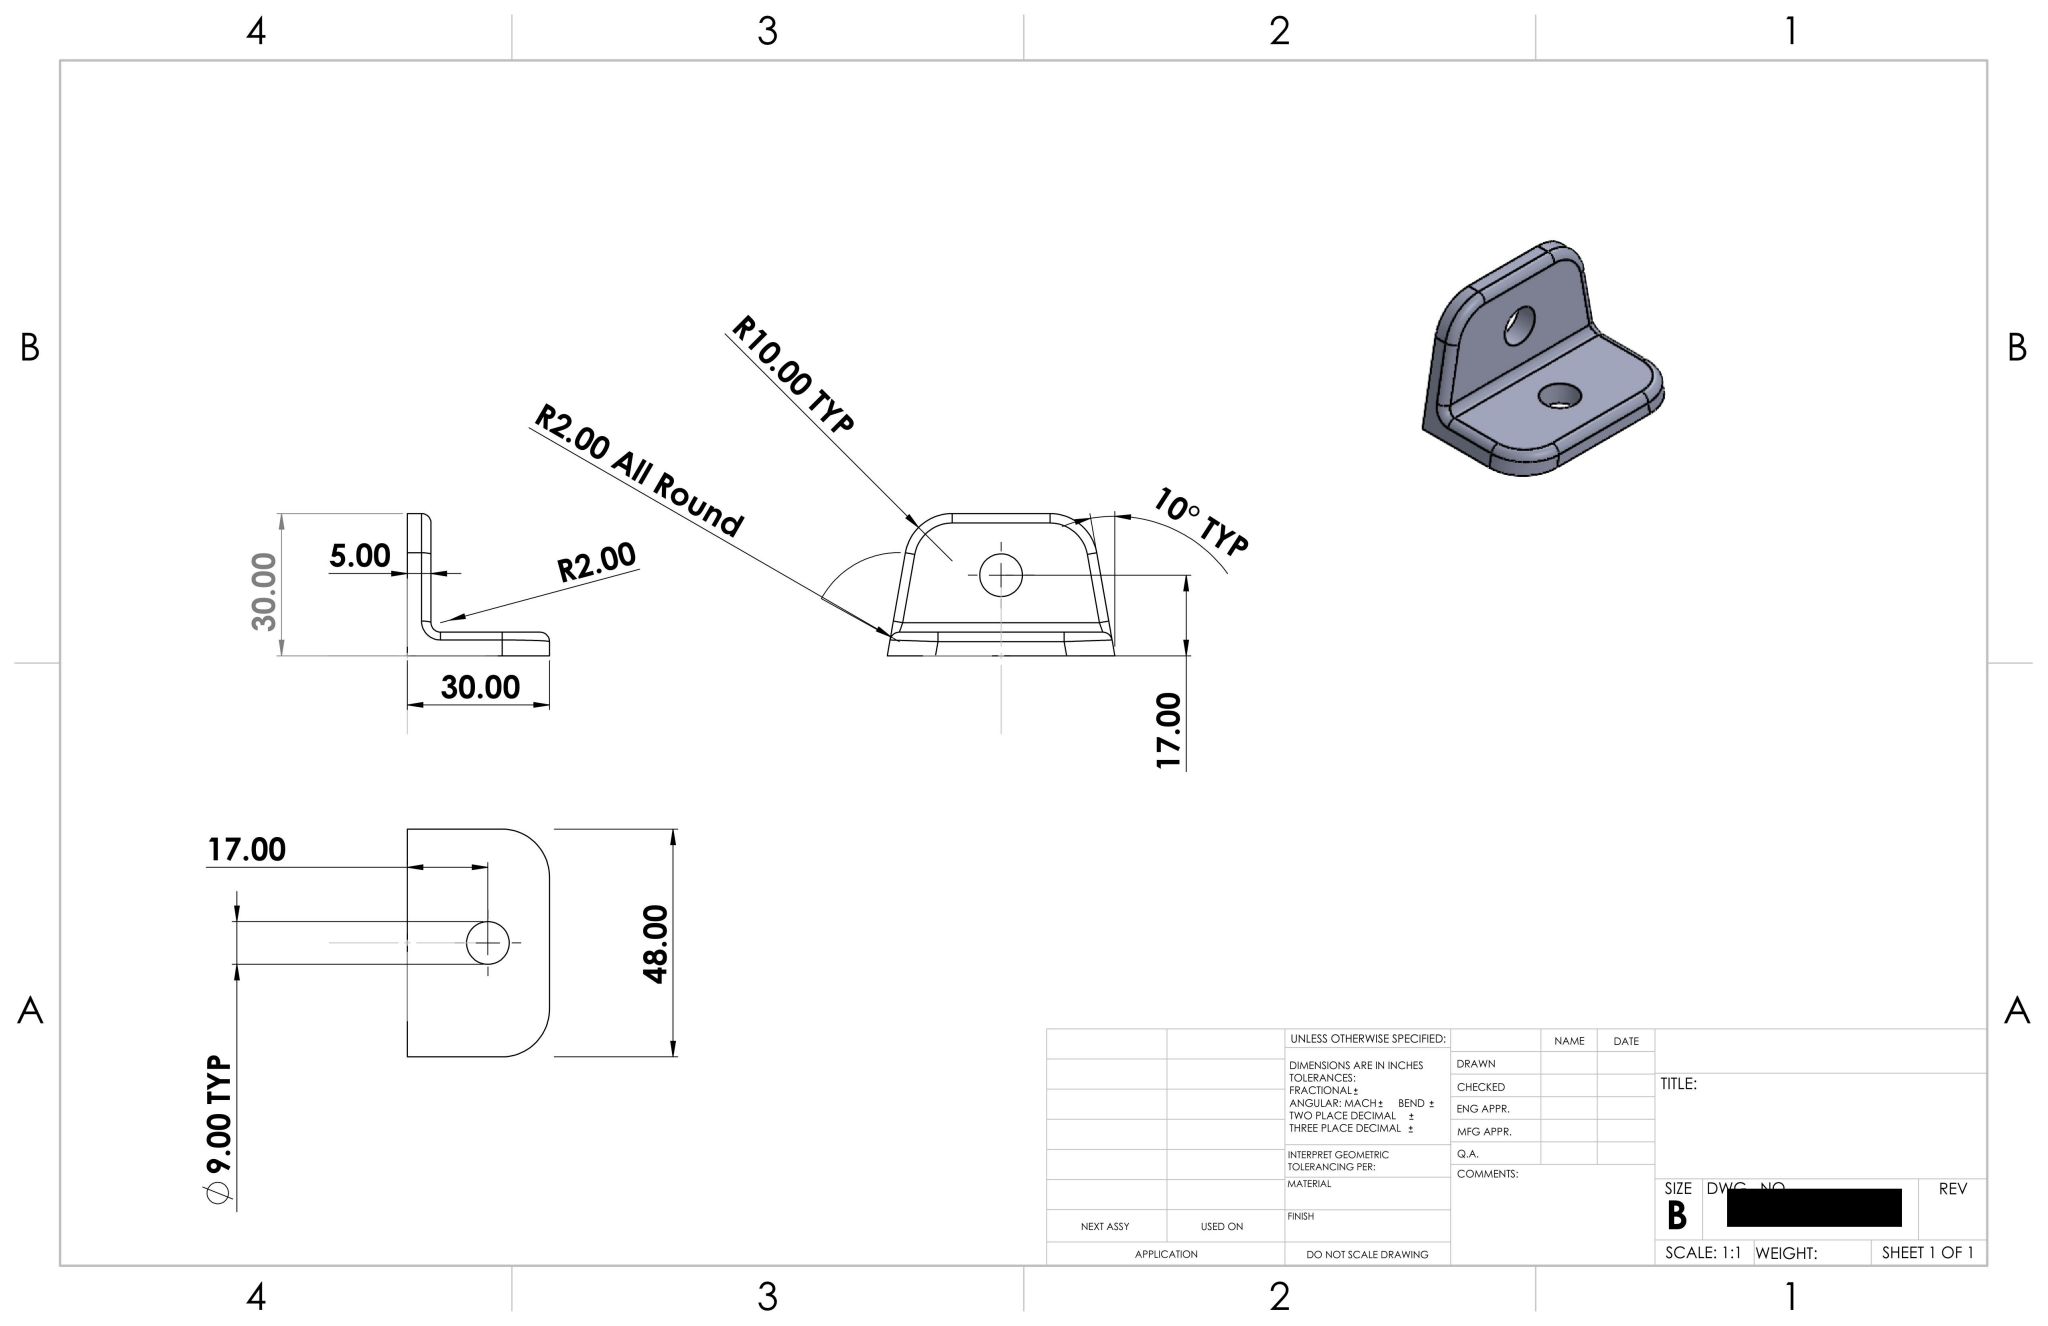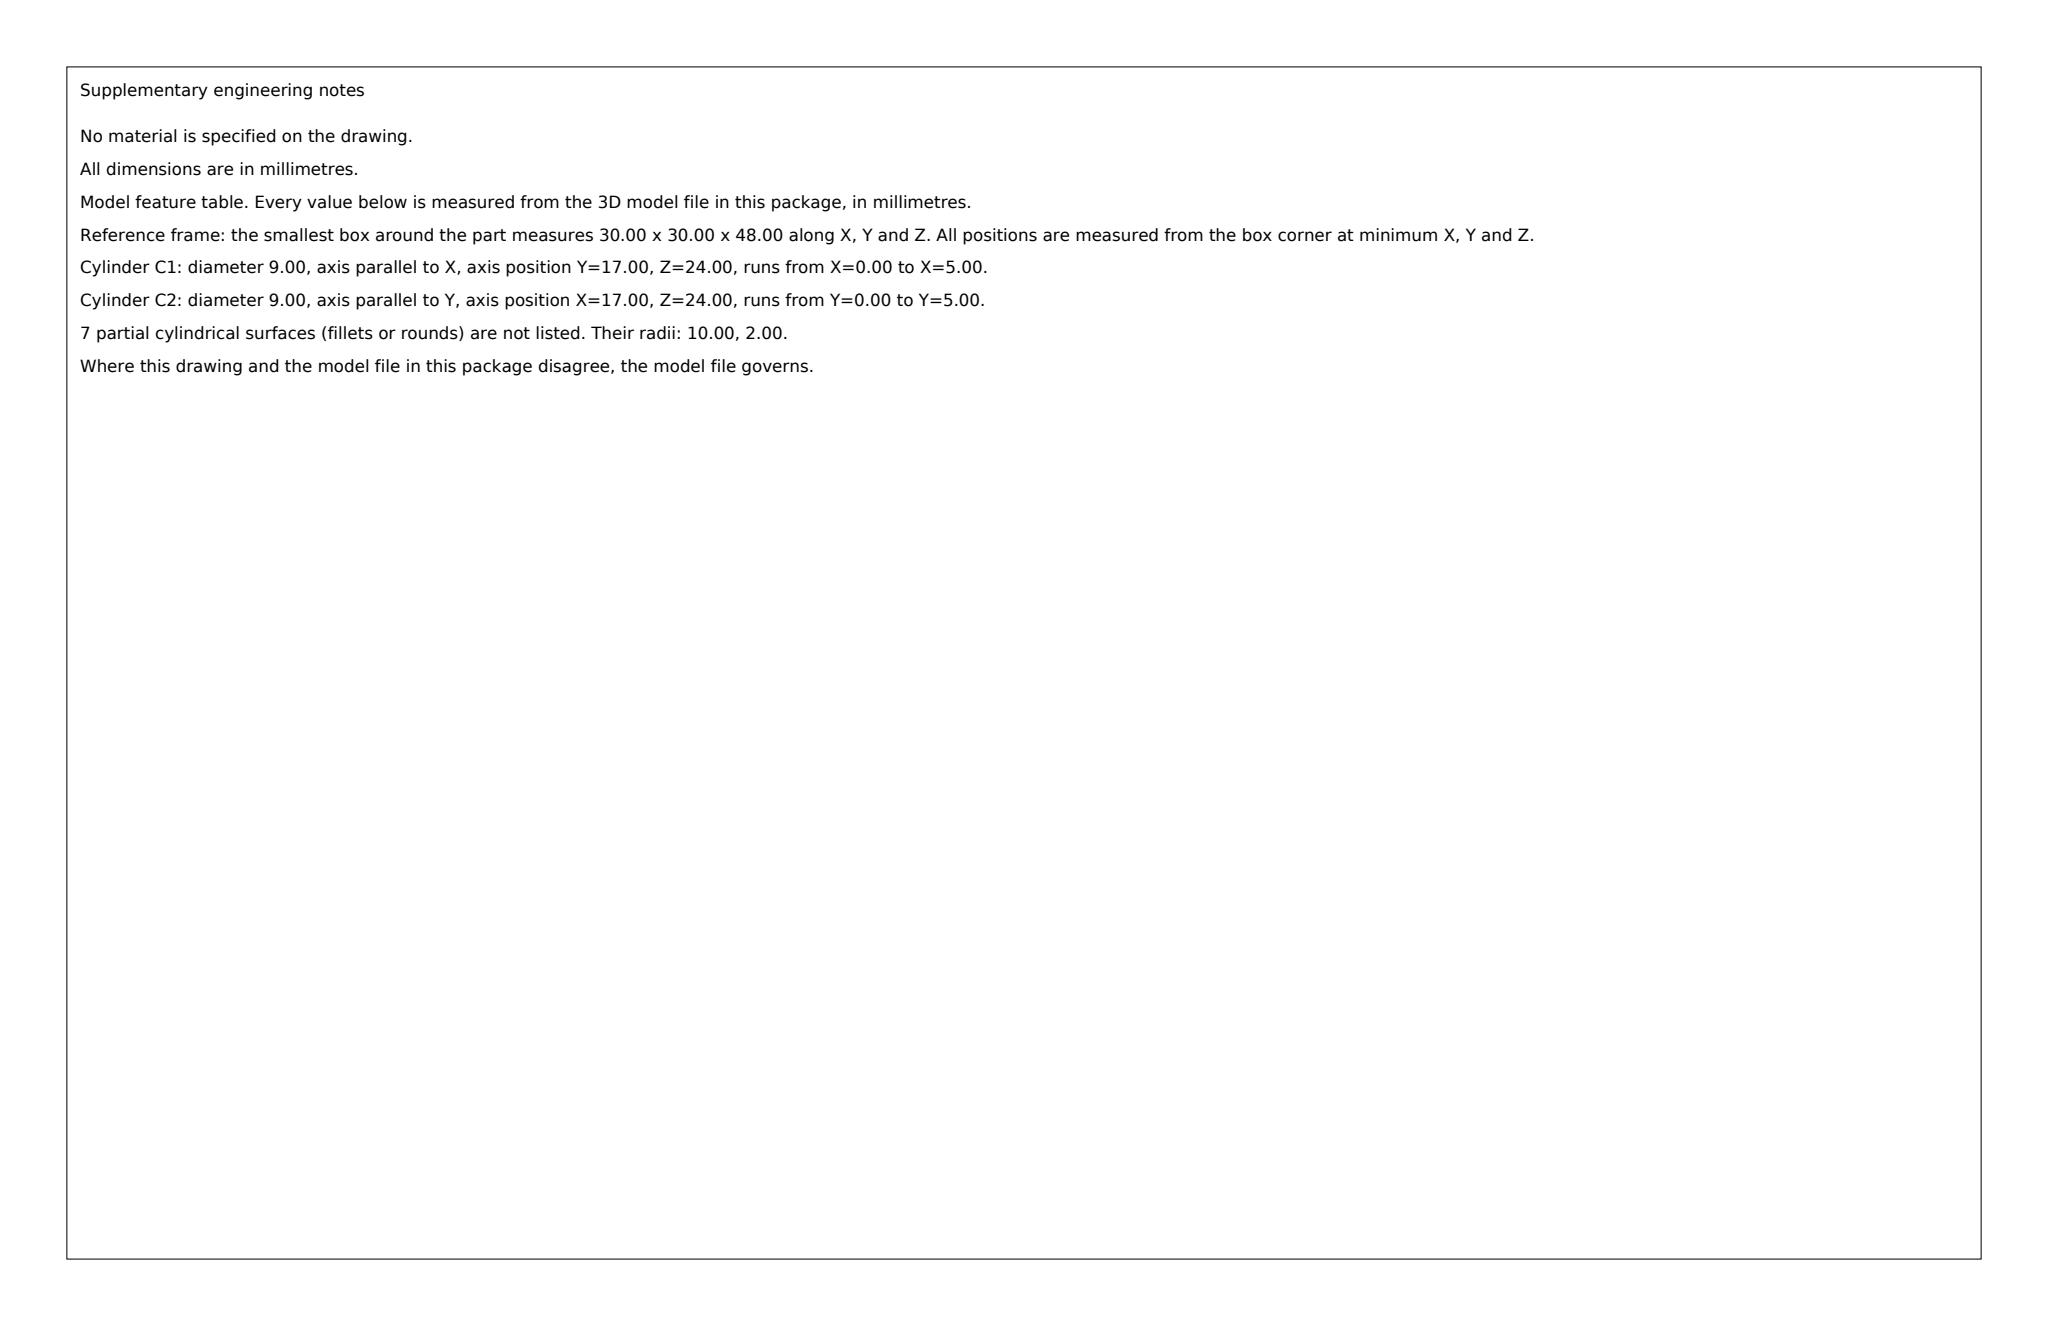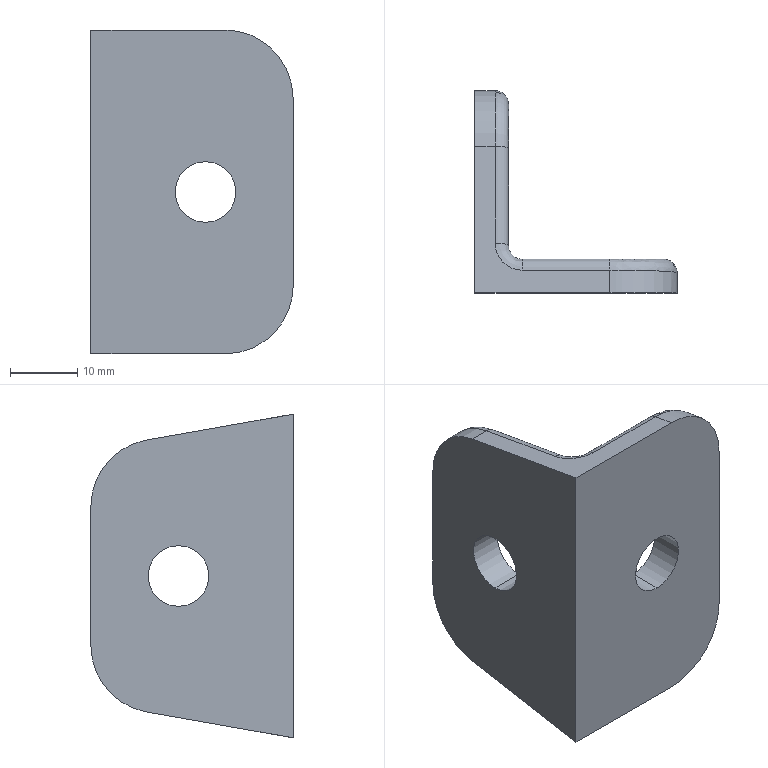Part | SolidWorks | mm | 1 solid | 29 faces | box 30 x 30 x 48 mm | volume 11212 mm3 | cylinder 15 | plane 8 | spline 4 | torus 2 | commonest cylinder face diameters 4 x7 9 x4 20 x4